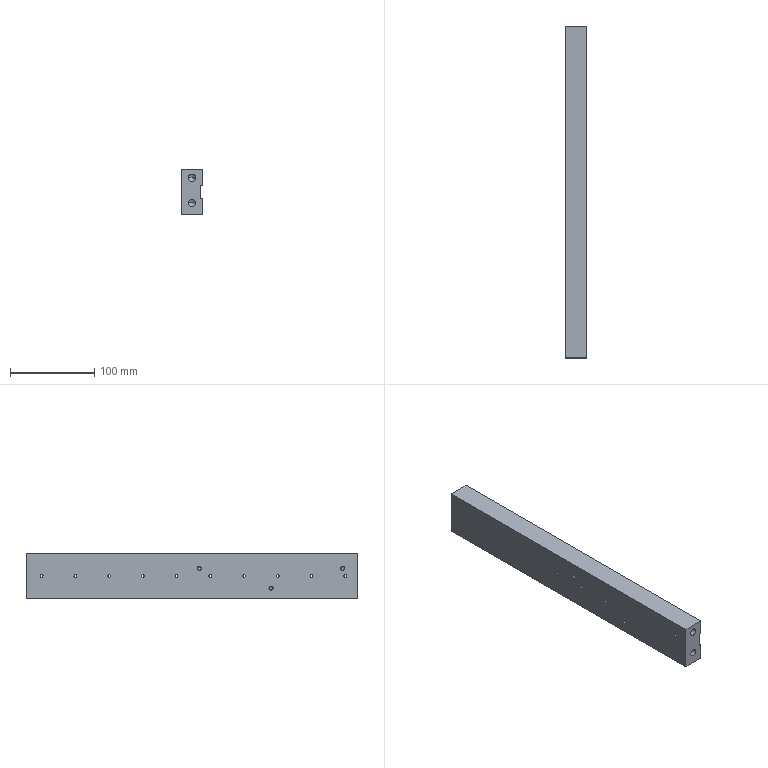Component | SolidWorks | FeedBarrelPistonBracket2-1 | 1 solid | 84 faces | box 25 x 393.5 x 54 mm | volume 502592 mm3 | cone 40 | cylinder 34 | plane 10 | commonest cylinder face diameters 3.3 x20 8.5 x8 4.2 x6
build123d program:
from build123d import *

# Parameters (mm, degrees)
SKETCH3_W                   = 25
SKETCH3_H                   = 54
BOSS_EXTRUDE1_DEPTH         = 393.5
M10_TAPPED_HOLE1_AT_2_COUNT = 2
M10_TAPPED_HOLE1_AT_2_PITCH = 30
SKETCH8_W                   = 393.5
SKETCH8_H                   = 16
CUT_EXTRUDE1_DEPTH          = 3
M4_TAPPED_HOLE1_D           = 3.3
M4_TAPPED_HOLE1_CSINK_D     = 4.05
M4_TAPPED_HOLE1_CSINK_ANGLE = 90
M5_TAPPED_HOLE2_D           = 4.2
M5_TAPPED_HOLE2_DEPTH       = 20
M5_TAPPED_HOLE2_CSINK_D     = 5.05
M5_TAPPED_HOLE2_CSINK_ANGLE = 90
M5_TAPPED_HOLE2_TIP         = 1.262


with BuildPart() as part:
    # Sketch3 → Boss-Extrude1 (new body)
    with BuildSketch(Plane.XY):
        with Locations((107.5, 27)):
            Rectangle(SKETCH3_W, SKETCH3_H)
    extrude(amount=BOSS_EXTRUDE1_DEPTH)

    # Sketch7 → M10 Tapped Hole1 (revolve, cut)
    with BuildSketch(Plane(origin=(107.5, 44, 0), x_dir=(0, 1, 0), z_dir=(1, 0, 0))):
        Polygon((0, 0), (0, 32.554), (4.25, 30), (4.25, 0), align=None)
    m10_tapped_hole1 = revolve(axis=Axis((107.5, 44, -6.35), (0, 0, 1)), mode=Mode.SUBTRACT)

    # M10 Tapped Hole1 at 2: M10 Tapped Hole1 ×2
    with Locations(*[(0, -i * M10_TAPPED_HOLE1_AT_2_PITCH, 0) for i in range(1, M10_TAPPED_HOLE1_AT_2_COUNT)]):
        add(m10_tapped_hole1, mode=Mode.SUBTRACT)

    # Mirror1: M10 Tapped Hole1 across plane
    add(m10_tapped_hole1.mirror(Plane(origin=(0, 0, 196.75), x_dir=(1, 0, 0), z_dir=(0, 0, -1))), mode=Mode.SUBTRACT)

    # Mirror1 copy 1 sketch → Mirror1 copy 1 (revolve, cut)
    with BuildSketch(Plane(origin=(107.5, 14, 393.5), x_dir=(0, 1, 0), z_dir=(1, 0, 0))):
        Polygon((0, 0), (0, -32.554), (4.25, -30), (4.25, 0), align=None)
    revolve(axis=Axis((107.5, 14, 399.85), (0, 0, 1)), mode=Mode.SUBTRACT)

    # Sketch8 → Cut-Extrude1 (cut)
    with BuildSketch(Plane(origin=(120, 0, 0), x_dir=(0, 0, -1), z_dir=(1, 0, 0))):
        with Locations((-196.75, 27)):
            Rectangle(SKETCH8_W, SKETCH8_H)
    extrude(amount=-CUT_EXTRUDE1_DEPTH, mode=Mode.SUBTRACT)

    # M4 Tapped Hole1 (through all)
    with Locations(Plane(origin=(117, 0, 0), x_dir=(0, 0, -1), z_dir=(1, 0, 0))):
        with Locations((-378.5, 27), (-18.5, 27), (-58.5, 27), (-98.5, 27), (-138.5, 27), (-178.5, 27), (-218.5, 27), (-258.5, 27), (-298.5, 27), (-338.5, 27)):
            CounterSinkHole(M4_TAPPED_HOLE1_D / 2, M4_TAPPED_HOLE1_CSINK_D / 2, counter_sink_angle=M4_TAPPED_HOLE1_CSINK_ANGLE)

    # M5 Tapped Hole2
    with Locations(Plane.ZY.offset(-95)):
        with Locations((205.5, 36), (375.5, 36), (290.5, 12.5)):
            CounterSinkHole(M5_TAPPED_HOLE2_D / 2, M5_TAPPED_HOLE2_CSINK_D / 2, depth=M5_TAPPED_HOLE2_DEPTH, counter_sink_angle=M5_TAPPED_HOLE2_CSINK_ANGLE)
            with Locations((0, 0, -(M5_TAPPED_HOLE2_DEPTH + M5_TAPPED_HOLE2_TIP / 2))):  # 118° drill point
                Cone(0, M5_TAPPED_HOLE2_D / 2, M5_TAPPED_HOLE2_TIP, mode=Mode.SUBTRACT)


solid = part.part

# Placed as in the assembly
solid = solid.moved(Location((-718.446, 245.849, 409.168), (90, 0, 0)))